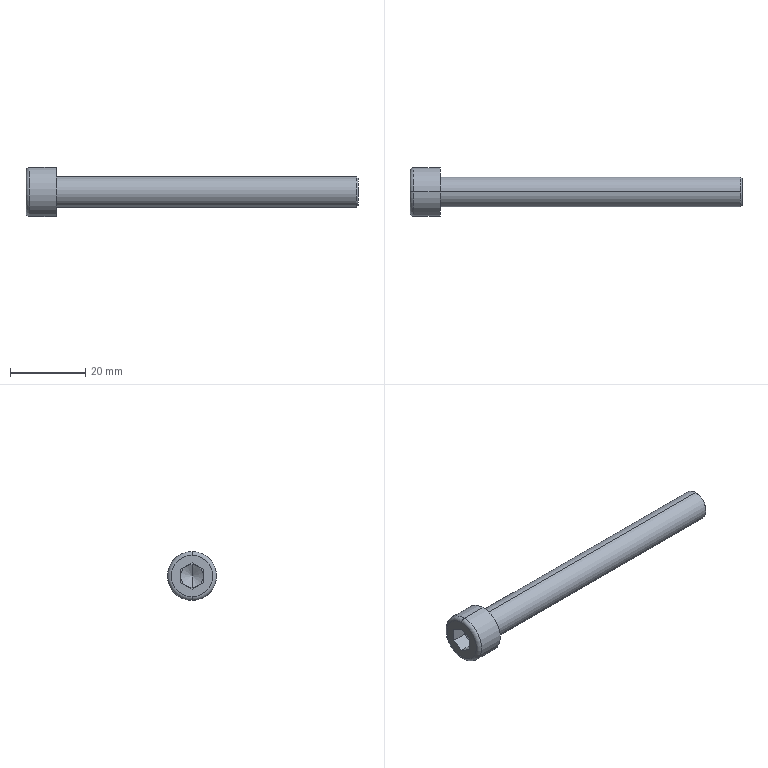Component | SolidWorks | M8X80-2 | 1 solid | 25 faces | box 88 x 13 x 13 mm | volume 4932 mm3 | plane 15 | cone 4 | cylinder 4 | torus 2 | commonest cylinder face diameters 8 x2 13 x2
build123d program:
from build123d import *

# Parameters (mm, degrees)
SKETCH1_R           = 6.5
BASEHEAD_DEPTH      = 8
SKETCH2_R           = 4
BASEBODY_DEPTH      = 80
HEXAGONSOCKET_DEPTH = 4
TOPFILLET_R         = 1
CHAMFER1_SIZE       = 0.4


with BuildPart() as part:
    # Sketch1 → BaseHead (new body)
    with BuildSketch(Plane(origin=(0, 0, 0), x_dir=(0, 0, -1), z_dir=(1, 0, 0))):
        Circle(SKETCH1_R)
    extrude(amount=BASEHEAD_DEPTH)

    # Sketch2 → BaseBody (add)
    with BuildSketch(Plane(origin=(8, 0, 0), x_dir=(0, 0, -1), z_dir=(1, 0, 0))):
        Circle(SKETCH2_R)
    extrude(amount=BASEBODY_DEPTH)

    # Sketch3 → HexagonSocket (cut)
    with BuildSketch(Plane(origin=(0, 0, 0), x_dir=(0, 0, -1), z_dir=(1, 0, 0))):
        Polygon((3.464, 0), (1.732, 3), (-1.732, 3), (-3.464, 0), (-1.732, -3), (1.732, -3), align=None)
    extrude(amount=HEXAGONSOCKET_DEPTH, mode=Mode.SUBTRACT)

    # Sketch4 → Cut-Revolve1 (revolve, cut)
    with BuildSketch(Plane(origin=(-4.196, 0.75, 0), x_dir=(-1, 0, 0), z_dir=(0, 0, 1)), mode=Mode.PRIVATE) as cut_revolve1_sk:
        Polygon((-8.196, 3.75), (-9.928, 0.75), (-8.196, 0.75), align=None)
    revolve(cut_revolve1_sk.sketch.rotate(Axis((0.839, 0, 0), (-1, 0, 0)), 90), axis=Axis((0.839, 0, 0), (-1, 0, 0)), mode=Mode.SUBTRACT)

    # TopFillet
    topfillet_edges = [part.edges().sort_by_distance(p)[0] for p in [
        (0, 0, 6.5),
    ]]
    fillet(topfillet_edges, radius=TOPFILLET_R)

    # Chamfer1
    chamfer1_edges = [part.edges().sort_by_distance(p)[0] for p in [
        (88, 0, 4),
    ]]
    chamfer(chamfer1_edges, length=CHAMFER1_SIZE)


solid = part.part

# Placed as in the assembly
solid = solid.moved(Location((-198, 1239.5, 160), (0, 0, 0)))
STEP:
#1=COLOUR_RGB('',0.7922,0.8196,0.9333);
#2=FILL_AREA_STYLE_COLOUR('',#1);
#3=FILL_AREA_STYLE('',(#2));
#4=SURFACE_STYLE_FILL_AREA(#3);
#5=SURFACE_SIDE_STYLE('',(#4));
#6=SURFACE_STYLE_USAGE(.BOTH.,#5);
#7=PRESENTATION_STYLE_ASSIGNMENT((#6));
#8=CARTESIAN_POINT('',(-4.331,48.799,6.157));
#9=VERTEX_POINT('',#8);
#10=CARTESIAN_POINT('',(-4.331,48.799,6.441));
#11=VERTEX_POINT('',#10);
#12=CARTESIAN_POINT('',(-4.331,48.799,6.299));
#13=DIRECTION('',(1.,0.,0.));
#14=DIRECTION('',(0.,0.,-1.));
#15=AXIS2_PLACEMENT_3D('',#12,#13,#14);
#16=CIRCLE('',#15,0.1417);
#17=EDGE_CURVE('',#9,#11,#16,.T.);
#18=ORIENTED_EDGE('',*,*,#17,.F.);
#19=CARTESIAN_POINT('',(-4.346,48.799,6.142));
#20=VERTEX_POINT('',#19);
#21=CARTESIAN_POINT('',(-4.331,48.799,6.157));
#22=DIRECTION('',(-0.7071,0.,-0.7071));
#23=VECTOR('',#22,39.37);
#24=LINE('',#21,#23);
#25=EDGE_CURVE('',#9,#20,#24,.T.);
#26=ORIENTED_EDGE('',*,*,#25,.T.);
#27=CARTESIAN_POINT('',(-4.346,48.799,6.457));
#28=VERTEX_POINT('',#27);
#29=CARTESIAN_POINT('',(-4.346,48.799,6.299));
#30=DIRECTION('',(-1.,0.,0.));
#31=DIRECTION('',(0.,0.,-1.));
#32=AXIS2_PLACEMENT_3D('',#29,#30,#31);
#33=CIRCLE('',#32,0.1575);
#34=EDGE_CURVE('',#28,#20,#33,.T.);
#35=ORIENTED_EDGE('',*,*,#34,.F.);
#36=CARTESIAN_POINT('',(-4.331,48.799,6.441));
#37=DIRECTION('',(-0.7071,0.,0.7071));
#38=VECTOR('',#37,39.37);
#39=LINE('',#36,#38);
#40=EDGE_CURVE('',#11,#28,#39,.T.);
#41=ORIENTED_EDGE('',*,*,#40,.F.);
#42=EDGE_LOOP('',(#18,#26,#35,#41));
#43=FACE_OUTER_BOUND('',#42,.T.);
#44=CARTESIAN_POINT('',(-4.331,48.799,6.299));
#45=DIRECTION('',(-1.,0.,0.));
#46=DIRECTION('',(0.,0.,1.));
#47=AXIS2_PLACEMENT_3D('',#44,#45,#46);
#48=CONICAL_SURFACE('',#47,0.1417,0.7854);
#49=ADVANCED_FACE('',(#43),#48,.T.);
#50=CARTESIAN_POINT('',(-7.795,48.799,6.516));
#51=VERTEX_POINT('',#50);
#52=CARTESIAN_POINT('',(-7.795,48.799,6.083));
#53=VERTEX_POINT('',#52);
#54=CARTESIAN_POINT('',(-7.795,48.799,6.299));
#55=DIRECTION('',(-1.,0.,0.));
#56=DIRECTION('',(0.,0.,-1.));
#57=AXIS2_PLACEMENT_3D('',#54,#55,#56);
#58=CIRCLE('',#57,0.2165);
#59=EDGE_CURVE('',#51,#53,#58,.T.);
#60=ORIENTED_EDGE('',*,*,#59,.F.);
#61=CARTESIAN_POINT('',(-7.756,48.799,6.555));
#62=VERTEX_POINT('',#61);
#63=CARTESIAN_POINT('',(-7.756,48.799,6.516));
#64=DIRECTION('',(0.,1.,-0.));
#65=DIRECTION('',(0.,0.,1.));
#66=AXIS2_PLACEMENT_3D('',#63,#64,#65);
#67=CIRCLE('',#66,0.03937);
#68=EDGE_CURVE('',#51,#62,#67,.T.);
#69=ORIENTED_EDGE('',*,*,#68,.T.);
#70=CARTESIAN_POINT('',(-7.756,48.799,6.043));
#71=VERTEX_POINT('',#70);
#72=CARTESIAN_POINT('',(-7.756,48.799,6.299));
#73=DIRECTION('',(1.,0.,0.));
#74=DIRECTION('',(0.,0.,-1.));
#75=AXIS2_PLACEMENT_3D('',#72,#73,#74);
#76=CIRCLE('',#75,0.2559);
#77=EDGE_CURVE('',#71,#62,#76,.T.);
#78=ORIENTED_EDGE('',*,*,#77,.F.);
#79=CARTESIAN_POINT('',(-7.756,48.799,6.083));
#80=DIRECTION('',(0.,-1.,0.));
#81=DIRECTION('',(0.,0.,-1.));
#82=AXIS2_PLACEMENT_3D('',#79,#80,#81);
#83=CIRCLE('',#82,0.03937);
#84=EDGE_CURVE('',#53,#71,#83,.T.);
#85=ORIENTED_EDGE('',*,*,#84,.F.);
#86=EDGE_LOOP('',(#60,#69,#78,#85));
#87=FACE_OUTER_BOUND('',#86,.T.);
#88=CARTESIAN_POINT('',(-7.756,48.799,6.299));
#89=DIRECTION('',(1.,0.,0.));
#90=DIRECTION('',(0.,0.,-1.));
#91=AXIS2_PLACEMENT_3D('',#88,#89,#90);
#92=TOROIDAL_SURFACE('',#91,0.2165,0.03937);
#93=ADVANCED_FACE('',(#87),#92,.T.);
#94=CARTESIAN_POINT('',(-7.57,48.799,6.299));
#95=VERTEX_POINT('',#94);
#96=CARTESIAN_POINT('',(-7.638,48.799,6.417));
#97=VERTEX_POINT('',#96);
#98=CARTESIAN_POINT('',(-7.638,48.799,6.417));
#99=DIRECTION('',(-0.5,0.,0.866));
#100=VECTOR('',#99,39.37);
#101=LINE('',#98,#100);
#102=EDGE_CURVE('',#95,#97,#101,.T.);
#103=ORIENTED_EDGE('',*,*,#102,.F.);
#104=CARTESIAN_POINT('',(-7.638,48.799,6.181));
#105=VERTEX_POINT('',#104);
#106=CARTESIAN_POINT('',(-7.638,48.799,6.181));
#107=DIRECTION('',(-0.5,0.,-0.866));
#108=VECTOR('',#107,39.37);
#109=LINE('',#106,#108);
#110=EDGE_CURVE('',#95,#105,#109,.T.);
#111=ORIENTED_EDGE('',*,*,#110,.T.);
#112=CARTESIAN_POINT('',(-7.638,48.74,6.197));
#113=VERTEX_POINT('',#112);
#114=CARTESIAN_POINT('',(-7.638,48.799,6.299));
#115=DIRECTION('',(-1.,0.,0.));
#116=DIRECTION('',(0.,0.,-1.));
#117=AXIS2_PLACEMENT_3D('',#114,#115,#116);
#118=CIRCLE('',#117,0.1181);
#119=EDGE_CURVE('',#105,#113,#118,.T.);
#120=ORIENTED_EDGE('',*,*,#119,.T.);
#121=CARTESIAN_POINT('',(-7.638,48.681,6.299));
#122=VERTEX_POINT('',#121);
#123=CARTESIAN_POINT('',(-7.638,48.799,6.299));
#124=DIRECTION('',(-1.,0.,0.));
#125=DIRECTION('',(0.,0.,-1.));
#126=AXIS2_PLACEMENT_3D('',#123,#124,#125);
#127=CIRCLE('',#126,0.1181);
#128=EDGE_CURVE('',#113,#122,#127,.T.);
#129=ORIENTED_EDGE('',*,*,#128,.T.);
#130=CARTESIAN_POINT('',(-7.638,48.74,6.401));
#131=VERTEX_POINT('',#130);
#132=CARTESIAN_POINT('',(-7.638,48.799,6.299));
#133=DIRECTION('',(-1.,0.,0.));
#134=DIRECTION('',(0.,0.,-1.));
#135=AXIS2_PLACEMENT_3D('',#132,#133,#134);
#136=CIRCLE('',#135,0.1181);
#137=EDGE_CURVE('',#122,#131,#136,.T.);
#138=ORIENTED_EDGE('',*,*,#137,.T.);
#139=CARTESIAN_POINT('',(-7.638,48.799,6.299));
#140=DIRECTION('',(-1.,0.,0.));
#141=DIRECTION('',(0.,0.,-1.));
#142=AXIS2_PLACEMENT_3D('',#139,#140,#141);
#143=CIRCLE('',#142,0.1181);
#144=EDGE_CURVE('',#131,#97,#143,.T.);
#145=ORIENTED_EDGE('',*,*,#144,.T.);
#146=EDGE_LOOP('',(#103,#111,#120,#129,#138,#145));
#147=FACE_OUTER_BOUND('',#146,.T.);
#148=CARTESIAN_POINT('',(-7.638,48.799,6.299));
#149=DIRECTION('',(-1.,0.,0.));
#150=DIRECTION('',(0.,0.,1.));
#151=AXIS2_PLACEMENT_3D('',#148,#149,#150);
#152=CONICAL_SURFACE('',#151,0.1181,1.047);
#153=ADVANCED_FACE('',(#147),#152,.F.);
#154=ORIENTED_EDGE('',*,*,#34,.T.);
#155=CARTESIAN_POINT('',(-7.48,48.799,6.142));
#156=VERTEX_POINT('',#155);
#157=CARTESIAN_POINT('',(-4.331,48.799,6.142));
#158=DIRECTION('',(-1.,0.,0.));
#159=VECTOR('',#158,39.37);
#160=LINE('',#157,#159);
#161=EDGE_CURVE('',#20,#156,#160,.T.);
#162=ORIENTED_EDGE('',*,*,#161,.T.);
#163=CARTESIAN_POINT('',(-7.48,48.799,6.457));
#164=VERTEX_POINT('',#163);
#165=CARTESIAN_POINT('',(-7.48,48.799,6.299));
#166=DIRECTION('',(1.,0.,0.));
#167=DIRECTION('',(0.,0.,-1.));
#168=AXIS2_PLACEMENT_3D('',#165,#166,#167);
#169=CIRCLE('',#168,0.1575);
#170=EDGE_CURVE('',#156,#164,#169,.T.);
#171=ORIENTED_EDGE('',*,*,#170,.T.);
#172=CARTESIAN_POINT('',(-4.331,48.799,6.457));
#173=DIRECTION('',(-1.,0.,0.));
#174=VECTOR('',#173,39.37);
#175=LINE('',#172,#174);
#176=EDGE_CURVE('',#28,#164,#175,.T.);
#177=ORIENTED_EDGE('',*,*,#176,.F.);
#178=EDGE_LOOP('',(#154,#162,#171,#177));
#179=FACE_OUTER_BOUND('',#178,.T.);
#180=CARTESIAN_POINT('',(-4.331,48.799,6.299));
#181=DIRECTION('',(-1.,0.,0.));
#182=DIRECTION('',(0.,0.,1.));
#183=AXIS2_PLACEMENT_3D('',#180,#181,#182);
#184=CYLINDRICAL_SURFACE('',#183,0.1575);
#185=ADVANCED_FACE('',(#179),#184,.T.);
#186=CARTESIAN_POINT('',(-7.48,48.799,6.043));
#187=VERTEX_POINT('',#186);
#188=CARTESIAN_POINT('',(-7.48,48.799,6.555));
#189=VERTEX_POINT('',#188);
#190=CARTESIAN_POINT('',(-7.48,48.799,6.299));
#191=DIRECTION('',(1.,0.,0.));
#192=DIRECTION('',(0.,0.,-1.));
#193=AXIS2_PLACEMENT_3D('',#190,#191,#192);
#194=CIRCLE('',#193,0.2559);
#195=EDGE_CURVE('',#187,#189,#194,.T.);
#196=ORIENTED_EDGE('',*,*,#195,.F.);
#197=CARTESIAN_POINT('',(-7.48,48.799,6.043));
#198=DIRECTION('',(-1.,0.,0.));
#199=VECTOR('',#198,39.37);
#200=LINE('',#197,#199);
#201=EDGE_CURVE('',#187,#71,#200,.T.);
#202=ORIENTED_EDGE('',*,*,#201,.T.);
#203=ORIENTED_EDGE('',*,*,#77,.T.);
#204=CARTESIAN_POINT('',(-7.48,48.799,6.555));
#205=DIRECTION('',(-1.,0.,0.));
#206=VECTOR('',#205,39.37);
#207=LINE('',#204,#206);
#208=EDGE_CURVE('',#189,#62,#207,.T.);
#209=ORIENTED_EDGE('',*,*,#208,.F.);
#210=EDGE_LOOP('',(#196,#202,#203,#209));
#211=FACE_OUTER_BOUND('',#210,.T.);
#212=CARTESIAN_POINT('',(-7.48,48.799,6.299));
#213=DIRECTION('',(-1.,0.,0.));
#214=DIRECTION('',(0.,0.,1.));
#215=AXIS2_PLACEMENT_3D('',#212,#213,#214);
#216=CYLINDRICAL_SURFACE('',#215,0.2559);
#217=ADVANCED_FACE('',(#211),#216,.T.);
#218=ORIENTED_EDGE('',*,*,#128,.F.);
#219=CARTESIAN_POINT('',(-7.638,48.681,6.231));
#220=VERTEX_POINT('',#219);
#221=CARTESIAN_POINT('',(-7.638,48.681,6.231));
#222=DIRECTION('',(0.,0.866,-0.5));
#223=VECTOR('',#222,39.37);
#224=LINE('',#221,#223);
#225=EDGE_CURVE('',#220,#113,#224,.T.);
#226=ORIENTED_EDGE('',*,*,#225,.F.);
#227=CARTESIAN_POINT('',(-7.638,48.681,6.367));
#228=DIRECTION('',(0.,-0.,-1.));
#229=VECTOR('',#228,39.37);
#230=LINE('',#227,#229);
#231=EDGE_CURVE('',#122,#220,#230,.T.);
#232=ORIENTED_EDGE('',*,*,#231,.F.);
#233=EDGE_LOOP('',(#218,#226,#232));
#234=FACE_OUTER_BOUND('',#233,.T.);
#235=CARTESIAN_POINT('',(-7.638,48.799,6.163));
#236=DIRECTION('',(1.,0.,0.));
#237=DIRECTION('',(0.,0.,-1.));
#238=AXIS2_PLACEMENT_3D('',#235,#236,#237);
#239=PLANE('',#238);
#240=ADVANCED_FACE('',(#234),#239,.F.);
#241=ORIENTED_EDGE('',*,*,#137,.F.);
#242=CARTESIAN_POINT('',(-7.638,48.681,6.367));
#243=VERTEX_POINT('',#242);
#244=CARTESIAN_POINT('',(-7.638,48.681,6.367));
#245=DIRECTION('',(0.,-0.,-1.));
#246=VECTOR('',#245,39.37);
#247=LINE('',#244,#246);
#248=EDGE_CURVE('',#243,#122,#247,.T.);
#249=ORIENTED_EDGE('',*,*,#248,.F.);
#250=CARTESIAN_POINT('',(-7.638,48.799,6.436));
#251=DIRECTION('',(0.,-0.866,-0.5));
#252=VECTOR('',#251,39.37);
#253=LINE('',#250,#252);
#254=EDGE_CURVE('',#131,#243,#253,.T.);
#255=ORIENTED_EDGE('',*,*,#254,.F.);
#256=EDGE_LOOP('',(#241,#249,#255));
#257=FACE_OUTER_BOUND('',#256,.T.);
#258=CARTESIAN_POINT('',(-7.638,48.799,6.163));
#259=DIRECTION('',(1.,0.,0.));
#260=DIRECTION('',(0.,0.,-1.));
#261=AXIS2_PLACEMENT_3D('',#258,#259,#260);
#262=PLANE('',#261);
#263=ADVANCED_FACE('',(#257),#262,.F.);
#264=ORIENTED_EDGE('',*,*,#144,.F.);
#265=CARTESIAN_POINT('',(-7.638,48.799,6.436));
#266=VERTEX_POINT('',#265);
#267=CARTESIAN_POINT('',(-7.638,48.799,6.436));
#268=DIRECTION('',(0.,-0.866,-0.5));
#269=VECTOR('',#268,39.37);
#270=LINE('',#267,#269);
#271=EDGE_CURVE('',#266,#131,#270,.T.);
#272=ORIENTED_EDGE('',*,*,#271,.F.);
#273=CARTESIAN_POINT('',(-7.638,48.858,6.401));
#274=VERTEX_POINT('',#273);
#275=CARTESIAN_POINT('',(-7.638,48.917,6.367));
#276=DIRECTION('',(0.,-0.866,0.5));
#277=VECTOR('',#276,39.37);
#278=LINE('',#275,#277);
#279=EDGE_CURVE('',#274,#266,#278,.T.);
#280=ORIENTED_EDGE('',*,*,#279,.F.);
#281=CARTESIAN_POINT('',(-7.638,48.799,6.299));
#282=DIRECTION('',(-1.,0.,0.));
#283=DIRECTION('',(0.,0.,-1.));
#284=AXIS2_PLACEMENT_3D('',#281,#282,#283);
#285=CIRCLE('',#284,0.1181);
#286=EDGE_CURVE('',#97,#274,#285,.T.);
#287=ORIENTED_EDGE('',*,*,#286,.F.);
#288=EDGE_LOOP('',(#264,#272,#280,#287));
#289=FACE_OUTER_BOUND('',#288,.T.);
#290=CARTESIAN_POINT('',(-7.638,48.799,6.163));
#291=DIRECTION('',(1.,0.,0.));
#292=DIRECTION('',(0.,0.,-1.));
#293=AXIS2_PLACEMENT_3D('',#290,#291,#292);
#294=PLANE('',#293);
#295=ADVANCED_FACE('',(#289),#294,.F.);
#296=CARTESIAN_POINT('',(-7.638,48.917,6.299));
#297=VERTEX_POINT('',#296);
#298=CARTESIAN_POINT('',(-7.638,48.799,6.299));
#299=DIRECTION('',(-1.,0.,0.));
#300=DIRECTION('',(0.,0.,-1.));
#301=AXIS2_PLACEMENT_3D('',#298,#299,#300);
#302=CIRCLE('',#301,0.1181);
#303=EDGE_CURVE('',#274,#297,#302,.T.);
#304=ORIENTED_EDGE('',*,*,#303,.F.);
#305=CARTESIAN_POINT('',(-7.638,48.917,6.367));
#306=VERTEX_POINT('',#305);
#307=CARTESIAN_POINT('',(-7.638,48.917,6.367));
#308=DIRECTION('',(0.,-0.866,0.5));
#309=VECTOR('',#308,39.37);
#310=LINE('',#307,#309);
#311=EDGE_CURVE('',#306,#274,#310,.T.);
#312=ORIENTED_EDGE('',*,*,#311,.F.);
#313=CARTESIAN_POINT('',(-7.638,48.917,6.231));
#314=DIRECTION('',(0.,0.,1.));
#315=VECTOR('',#314,39.37);
#316=LINE('',#313,#315);
#317=EDGE_CURVE('',#297,#306,#316,.T.);
#318=ORIENTED_EDGE('',*,*,#317,.F.);
#319=EDGE_LOOP('',(#304,#312,#318));
#320=FACE_OUTER_BOUND('',#319,.T.);
#321=CARTESIAN_POINT('',(-7.638,48.799,6.163));
#322=DIRECTION('',(1.,0.,0.));
#323=DIRECTION('',(0.,0.,-1.));
#324=AXIS2_PLACEMENT_3D('',#321,#322,#323);
#325=PLANE('',#324);
#326=ADVANCED_FACE('',(#320),#325,.F.);
#327=CARTESIAN_POINT('',(-7.638,48.858,6.197));
#328=VERTEX_POINT('',#327);
#329=CARTESIAN_POINT('',(-7.638,48.799,6.299));
#330=DIRECTION('',(1.,0.,0.));
#331=DIRECTION('',(0.,0.,-1.));
#332=AXIS2_PLACEMENT_3D('',#329,#330,#331);
#333=CIRCLE('',#332,0.1181);
#334=EDGE_CURVE('',#328,#297,#333,.T.);
#335=ORIENTED_EDGE('',*,*,#334,.T.);
#336=CARTESIAN_POINT('',(-7.638,48.917,6.231));
#337=VERTEX_POINT('',#336);
#338=CARTESIAN_POINT('',(-7.638,48.917,6.231));
#339=DIRECTION('',(0.,0.,1.));
#340=VECTOR('',#339,39.37);
#341=LINE('',#338,#340);
#342=EDGE_CURVE('',#337,#297,#341,.T.);
#343=ORIENTED_EDGE('',*,*,#342,.F.);
#344=CARTESIAN_POINT('',(-7.638,48.799,6.163));
#345=DIRECTION('',(0.,0.866,0.5));
#346=VECTOR('',#345,39.37);
#347=LINE('',#344,#346);
#348=EDGE_CURVE('',#328,#337,#347,.T.);
#349=ORIENTED_EDGE('',*,*,#348,.F.);
#350=EDGE_LOOP('',(#335,#343,#349));
#351=FACE_OUTER_BOUND('',#350,.T.);
#352=CARTESIAN_POINT('',(-7.638,48.799,6.163));
#353=DIRECTION('',(1.,0.,0.));
#354=DIRECTION('',(0.,0.,-1.));
#355=AXIS2_PLACEMENT_3D('',#352,#353,#354);
#356=PLANE('',#355);
#357=ADVANCED_FACE('',(#351),#356,.F.);
#358=CARTESIAN_POINT('',(-7.638,48.799,6.299));
#359=DIRECTION('',(-1.,0.,0.));
#360=DIRECTION('',(0.,0.,-1.));
#361=AXIS2_PLACEMENT_3D('',#358,#359,#360);
#362=CIRCLE('',#361,0.1181);
#363=EDGE_CURVE('',#328,#105,#362,.T.);
#364=ORIENTED_EDGE('',*,*,#363,.F.);
#365=CARTESIAN_POINT('',(-7.638,48.799,6.163));
#366=VERTEX_POINT('',#365);
#367=CARTESIAN_POINT('',(-7.638,48.799,6.163));
#368=DIRECTION('',(0.,0.866,0.5));
#369=VECTOR('',#368,39.37);
#370=LINE('',#367,#369);
#371=EDGE_CURVE('',#366,#328,#370,.T.);
#372=ORIENTED_EDGE('',*,*,#371,.F.);
#373=CARTESIAN_POINT('',(-7.638,48.681,6.231));
#374=DIRECTION('',(0.,0.866,-0.5));
#375=VECTOR('',#374,39.37);
#376=LINE('',#373,#375);
#377=EDGE_CURVE('',#113,#366,#376,.T.);
#378=ORIENTED_EDGE('',*,*,#377,.F.);
#379=ORIENTED_EDGE('',*,*,#119,.F.);
#380=EDGE_LOOP('',(#364,#372,#378,#379));
#381=FACE_OUTER_BOUND('',#380,.T.);
#382=CARTESIAN_POINT('',(-7.638,48.799,6.163));
#383=DIRECTION('',(1.,0.,0.));
#384=DIRECTION('',(0.,0.,-1.));
#385=AXIS2_PLACEMENT_3D('',#382,#383,#384);
#386=PLANE('',#385);
#387=ADVANCED_FACE('',(#381),#386,.F.);
#388=CARTESIAN_POINT('',(-7.795,48.799,6.299));
#389=DIRECTION('',(-1.,0.,0.));
#390=DIRECTION('',(0.,0.,-1.));
#391=AXIS2_PLACEMENT_3D('',#388,#389,#390);
#392=CIRCLE('',#391,0.2165);
#393=EDGE_CURVE('',#53,#51,#392,.T.);
#394=ORIENTED_EDGE('',*,*,#393,.T.);
#395=ORIENTED_EDGE('',*,*,#59,.T.);
#396=EDGE_LOOP('',(#394,#395));
#397=FACE_OUTER_BOUND('',#396,.T.);
#398=CARTESIAN_POINT('',(-7.795,48.681,6.231));
#399=VERTEX_POINT('',#398);
#400=CARTESIAN_POINT('',(-7.795,48.799,6.163));
#401=VERTEX_POINT('',#400);
#402=CARTESIAN_POINT('',(-7.795,48.681,6.231));
#403=DIRECTION('',(0.,0.866,-0.5));
#404=VECTOR('',#403,39.37);
#405=LINE('',#402,#404);
#406=EDGE_CURVE('',#399,#401,#405,.T.);
#407=ORIENTED_EDGE('',*,*,#406,.T.);
#408=CARTESIAN_POINT('',(-7.795,48.917,6.231));
#409=VERTEX_POINT('',#408);
#410=CARTESIAN_POINT('',(-7.795,48.799,6.163));
#411=DIRECTION('',(0.,0.866,0.5));
#412=VECTOR('',#411,39.37);
#413=LINE('',#410,#412);
#414=EDGE_CURVE('',#401,#409,#413,.T.);
#415=ORIENTED_EDGE('',*,*,#414,.T.);
#416=CARTESIAN_POINT('',(-7.795,48.917,6.367));
#417=VERTEX_POINT('',#416);
#418=CARTESIAN_POINT('',(-7.795,48.917,6.231));
#419=DIRECTION('',(0.,0.,1.));
#420=VECTOR('',#419,39.37);
#421=LINE('',#418,#420);
#422=EDGE_CURVE('',#409,#417,#421,.T.);
#423=ORIENTED_EDGE('',*,*,#422,.T.);
#424=CARTESIAN_POINT('',(-7.795,48.799,6.436));
#425=VERTEX_POINT('',#424);
#426=CARTESIAN_POINT('',(-7.795,48.917,6.367));
#427=DIRECTION('',(0.,-0.866,0.5));
#428=VECTOR('',#427,39.37);
#429=LINE('',#426,#428);
#430=EDGE_CURVE('',#417,#425,#429,.T.);
#431=ORIENTED_EDGE('',*,*,#430,.T.);
#432=CARTESIAN_POINT('',(-7.795,48.681,6.367));
#433=VERTEX_POINT('',#432);
#434=CARTESIAN_POINT('',(-7.795,48.799,6.436));
#435=DIRECTION('',(0.,-0.866,-0.5));
#436=VECTOR('',#435,39.37);
#437=LINE('',#434,#436);
#438=EDGE_CURVE('',#425,#433,#437,.T.);
#439=ORIENTED_EDGE('',*,*,#438,.T.);
#440=CARTESIAN_POINT('',(-7.795,48.681,6.367));
#441=DIRECTION('',(0.,-0.,-1.));
#442=VECTOR('',#441,39.37);
#443=LINE('',#440,#442);
#444=EDGE_CURVE('',#433,#399,#443,.T.);
#445=ORIENTED_EDGE('',*,*,#444,.T.);
#446=EDGE_LOOP('',(#407,#415,#423,#431,#439,#445));
#447=FACE_BOUND('',#446,.T.);
#448=CARTESIAN_POINT('',(-7.795,48.799,6.299));
#449=DIRECTION('',(1.,0.,0.));
#450=DIRECTION('',(0.,0.,-1.));
#451=AXIS2_PLACEMENT_3D('',#448,#449,#450);
#452=PLANE('',#451);
#453=ADVANCED_FACE('',(#397,#447),#452,.F.);
#454=CARTESIAN_POINT('',(-7.48,48.799,6.299));
#455=DIRECTION('',(1.,0.,0.));
#456=DIRECTION('',(0.,0.,-1.));
#457=AXIS2_PLACEMENT_3D('',#454,#455,#456);
#458=CIRCLE('',#457,0.2559);
#459=EDGE_CURVE('',#189,#187,#458,.T.);
#460=ORIENTED_EDGE('',*,*,#459,.T.);
#461=ORIENTED_EDGE('',*,*,#195,.T.);
#462=EDGE_LOOP('',(#460,#461));
#463=FACE_OUTER_BOUND('',#462,.T.);
#464=CARTESIAN_POINT('',(-7.48,48.799,6.299));
#465=DIRECTION('',(1.,0.,0.));
#466=DIRECTION('',(0.,0.,-1.));
#467=AXIS2_PLACEMENT_3D('',#464,#465,#466);
#468=CIRCLE('',#467,0.1575);
#469=EDGE_CURVE('',#164,#156,#468,.T.);
#470=ORIENTED_EDGE('',*,*,#469,.F.);
#471=ORIENTED_EDGE('',*,*,#170,.F.);
#472=EDGE_LOOP('',(#470,#471));
#473=FACE_BOUND('',#472,.T.);
#474=CARTESIAN_POINT('',(-7.48,48.799,6.299));
#475=DIRECTION('',(1.,0.,0.));
#476=DIRECTION('',(0.,0.,-1.));
#477=AXIS2_PLACEMENT_3D('',#474,#475,#476);
#478=PLANE('',#477);
#479=ADVANCED_FACE('',(#463,#473),#478,.T.);
#480=ORIENTED_EDGE('',*,*,#201,.F.);
#481=ORIENTED_EDGE('',*,*,#459,.F.);
#482=ORIENTED_EDGE('',*,*,#208,.T.);
#483=CARTESIAN_POINT('',(-7.756,48.799,6.299));
#484=DIRECTION('',(1.,0.,0.));
#485=DIRECTION('',(0.,0.,-1.));
#486=AXIS2_PLACEMENT_3D('',#483,#484,#485);
#487=CIRCLE('',#486,0.2559);
#488=EDGE_CURVE('',#62,#71,#487,.T.);
#489=ORIENTED_EDGE('',*,*,#488,.T.);
#490=EDGE_LOOP('',(#480,#481,#482,#489));
#491=FACE_OUTER_BOUND('',#490,.T.);
#492=CARTESIAN_POINT('',(-7.48,48.799,6.299));
#493=DIRECTION('',(-1.,0.,0.));
#494=DIRECTION('',(0.,0.,1.));
#495=AXIS2_PLACEMENT_3D('',#492,#493,#494);
#496=CYLINDRICAL_SURFACE('',#495,0.2559);
#497=ADVANCED_FACE('',(#491),#496,.T.);
#498=ORIENTED_EDGE('',*,*,#161,.F.);
#499=CARTESIAN_POINT('',(-4.346,48.799,6.299));
#500=DIRECTION('',(-1.,0.,0.));
#501=DIRECTION('',(0.,0.,-1.));
#502=AXIS2_PLACEMENT_3D('',#499,#500,#501);
#503=CIRCLE('',#502,0.1575);
#504=EDGE_CURVE('',#20,#28,#503,.T.);
#505=ORIENTED_EDGE('',*,*,#504,.T.);
#506=ORIENTED_EDGE('',*,*,#176,.T.);
#507=ORIENTED_EDGE('',*,*,#469,.T.);
#508=EDGE_LOOP('',(#498,#505,#506,#507));
#509=FACE_OUTER_BOUND('',#508,.T.);
#510=CARTESIAN_POINT('',(-4.331,48.799,6.299));
#511=DIRECTION('',(-1.,0.,0.));
#512=DIRECTION('',(0.,0.,1.));
#513=AXIS2_PLACEMENT_3D('',#510,#511,#512);
#514=CYLINDRICAL_SURFACE('',#513,0.1575);
#515=ADVANCED_FACE('',(#509),#514,.T.);
#516=CARTESIAN_POINT('',(-4.331,48.799,6.299));
#517=DIRECTION('',(1.,0.,0.));
#518=DIRECTION('',(0.,0.,-1.));
#519=AXIS2_PLACEMENT_3D('',#516,#517,#518);
#520=CIRCLE('',#519,0.1417);
#521=EDGE_CURVE('',#11,#9,#520,.T.);
#522=ORIENTED_EDGE('',*,*,#521,.T.);
#523=ORIENTED_EDGE('',*,*,#17,.T.);
#524=EDGE_LOOP('',(#522,#523));
#525=FACE_OUTER_BOUND('',#524,.T.);
#526=CARTESIAN_POINT('',(-4.331,48.799,6.299));
#527=DIRECTION('',(1.,0.,0.));
#528=DIRECTION('',(0.,0.,-1.));
#529=AXIS2_PLACEMENT_3D('',#526,#527,#528);
#530=PLANE('',#529);
#531=ADVANCED_FACE('',(#525),#530,.T.);
#532=ORIENTED_EDGE('',*,*,#406,.F.);
#533=CARTESIAN_POINT('',(-7.638,48.681,6.231));
#534=DIRECTION('',(-1.,0.,0.));
#535=VECTOR('',#534,39.37);
#536=LINE('',#533,#535);
#537=EDGE_CURVE('',#220,#399,#536,.T.);
#538=ORIENTED_EDGE('',*,*,#537,.F.);
#539=ORIENTED_EDGE('',*,*,#225,.T.);
#540=ORIENTED_EDGE('',*,*,#377,.T.);
#541=CARTESIAN_POINT('',(-7.638,48.799,6.163));
#542=DIRECTION('',(-1.,0.,0.));
#543=VECTOR('',#542,39.37);
#544=LINE('',#541,#543);
#545=EDGE_CURVE('',#366,#401,#544,.T.);
#546=ORIENTED_EDGE('',*,*,#545,.T.);
#547=EDGE_LOOP('',(#532,#538,#539,#540,#546));
#548=FACE_OUTER_BOUND('',#547,.T.);
#549=CARTESIAN_POINT('',(-7.638,48.681,6.231));
#550=DIRECTION('',(0.,0.5,0.866));
#551=DIRECTION('',(0.,-0.866,0.5));
#552=AXIS2_PLACEMENT_3D('',#549,#550,#551);
#553=PLANE('',#552);
#554=ADVANCED_FACE('',(#548),#553,.T.);
#555=ORIENTED_EDGE('',*,*,#414,.F.);
#556=ORIENTED_EDGE('',*,*,#545,.F.);
#557=ORIENTED_EDGE('',*,*,#371,.T.);
#558=ORIENTED_EDGE('',*,*,#348,.T.);
#559=CARTESIAN_POINT('',(-7.638,48.917,6.231));
#560=DIRECTION('',(-1.,0.,0.));
#561=VECTOR('',#560,39.37);
#562=LINE('',#559,#561);
#563=EDGE_CURVE('',#337,#409,#562,.T.);
#564=ORIENTED_EDGE('',*,*,#563,.T.);
#565=EDGE_LOOP('',(#555,#556,#557,#558,#564));
#566=FACE_OUTER_BOUND('',#565,.T.);
#567=CARTESIAN_POINT('',(-7.638,48.799,6.163));
#568=DIRECTION('',(0.,-0.5,0.866));
#569=DIRECTION('',(0.,-0.866,-0.5));
#570=AXIS2_PLACEMENT_3D('',#567,#568,#569);
#571=PLANE('',#570);
#572=ADVANCED_FACE('',(#566),#571,.T.);
#573=ORIENTED_EDGE('',*,*,#422,.F.);
#574=ORIENTED_EDGE('',*,*,#563,.F.);
#575=ORIENTED_EDGE('',*,*,#342,.T.);
#576=ORIENTED_EDGE('',*,*,#317,.T.);
#577=CARTESIAN_POINT('',(-7.638,48.917,6.367));
#578=DIRECTION('',(-1.,0.,0.));
#579=VECTOR('',#578,39.37);
#580=LINE('',#577,#579);
#581=EDGE_CURVE('',#306,#417,#580,.T.);
#582=ORIENTED_EDGE('',*,*,#581,.T.);
#583=EDGE_LOOP('',(#573,#574,#575,#576,#582));
#584=FACE_OUTER_BOUND('',#583,.T.);
#585=CARTESIAN_POINT('',(-7.638,48.917,6.231));
#586=DIRECTION('',(0.,-1.,0.));
#587=DIRECTION('',(0.,0.,-1.));
#588=AXIS2_PLACEMENT_3D('',#585,#586,#587);
#589=PLANE('',#588);
#590=ADVANCED_FACE('',(#584),#589,.T.);
#591=ORIENTED_EDGE('',*,*,#430,.F.);
#592=ORIENTED_EDGE('',*,*,#581,.F.);
#593=ORIENTED_EDGE('',*,*,#311,.T.);
#594=ORIENTED_EDGE('',*,*,#279,.T.);
#595=CARTESIAN_POINT('',(-7.638,48.799,6.436));
#596=DIRECTION('',(-1.,0.,0.));
#597=VECTOR('',#596,39.37);
#598=LINE('',#595,#597);
#599=EDGE_CURVE('',#266,#425,#598,.T.);
#600=ORIENTED_EDGE('',*,*,#599,.T.);
#601=EDGE_LOOP('',(#591,#592,#593,#594,#600));
#602=FACE_OUTER_BOUND('',#601,.T.);
#603=CARTESIAN_POINT('',(-7.638,48.917,6.367));
#604=DIRECTION('',(0.,-0.5,-0.866));
#605=DIRECTION('',(0.,0.866,-0.5));
#606=AXIS2_PLACEMENT_3D('',#603,#604,#605);
#607=PLANE('',#606);
#608=ADVANCED_FACE('',(#602),#607,.T.);
#609=ORIENTED_EDGE('',*,*,#438,.F.);
#610=ORIENTED_EDGE('',*,*,#599,.F.);
#611=ORIENTED_EDGE('',*,*,#271,.T.);
#612=ORIENTED_EDGE('',*,*,#254,.T.);
#613=CARTESIAN_POINT('',(-7.638,48.681,6.367));
#614=DIRECTION('',(-1.,0.,0.));
#615=VECTOR('',#614,39.37);
#616=LINE('',#613,#615);
#617=EDGE_CURVE('',#243,#433,#616,.T.);
#618=ORIENTED_EDGE('',*,*,#617,.T.);
#619=EDGE_LOOP('',(#609,#610,#611,#612,#618));
#620=FACE_OUTER_BOUND('',#619,.T.);
#621=CARTESIAN_POINT('',(-7.638,48.799,6.436));
#622=DIRECTION('',(0.,0.5,-0.866));
#623=DIRECTION('',(0.,0.866,0.5));
#624=AXIS2_PLACEMENT_3D('',#621,#622,#623);
#625=PLANE('',#624);
#626=ADVANCED_FACE('',(#620),#625,.T.);
#627=ORIENTED_EDGE('',*,*,#444,.F.);
#628=ORIENTED_EDGE('',*,*,#617,.F.);
#629=ORIENTED_EDGE('',*,*,#248,.T.);
#630=ORIENTED_EDGE('',*,*,#231,.T.);
#631=ORIENTED_EDGE('',*,*,#537,.T.);
#632=EDGE_LOOP('',(#627,#628,#629,#630,#631));
#633=FACE_OUTER_BOUND('',#632,.T.);
#634=CARTESIAN_POINT('',(-7.638,48.681,6.367));
#635=DIRECTION('',(0.,1.,-0.));
#636=DIRECTION('',(0.,0.,1.));
#637=AXIS2_PLACEMENT_3D('',#634,#635,#636);
#638=PLANE('',#637);
#639=ADVANCED_FACE('',(#633),#638,.T.);
#640=ORIENTED_EDGE('',*,*,#110,.F.);
#641=ORIENTED_EDGE('',*,*,#102,.T.);
#642=ORIENTED_EDGE('',*,*,#286,.T.);
#643=ORIENTED_EDGE('',*,*,#303,.T.);
#644=ORIENTED_EDGE('',*,*,#334,.F.);
#645=ORIENTED_EDGE('',*,*,#363,.T.);
#646=EDGE_LOOP('',(#640,#641,#642,#643,#644,#645));
#647=FACE_OUTER_BOUND('',#646,.T.);
#648=CARTESIAN_POINT('',(-7.638,48.799,6.299));
#649=DIRECTION('',(-1.,0.,0.));
#650=DIRECTION('',(0.,0.,1.));
#651=AXIS2_PLACEMENT_3D('',#648,#649,#650);
#652=CONICAL_SURFACE('',#651,0.1181,1.047);
#653=ADVANCED_FACE('',(#647),#652,.F.);
#654=ORIENTED_EDGE('',*,*,#68,.F.);
#655=ORIENTED_EDGE('',*,*,#393,.F.);
#656=ORIENTED_EDGE('',*,*,#84,.T.);
#657=ORIENTED_EDGE('',*,*,#488,.F.);
#658=EDGE_LOOP('',(#654,#655,#656,#657));
#659=FACE_OUTER_BOUND('',#658,.T.);
#660=CARTESIAN_POINT('',(-7.756,48.799,6.299));
#661=DIRECTION('',(1.,0.,0.));
#662=DIRECTION('',(0.,0.,-1.));
#663=AXIS2_PLACEMENT_3D('',#660,#661,#662);
#664=TOROIDAL_SURFACE('',#663,0.2165,0.03937);
#665=ADVANCED_FACE('',(#659),#664,.T.);
#666=ORIENTED_EDGE('',*,*,#25,.F.);
#667=ORIENTED_EDGE('',*,*,#521,.F.);
#668=ORIENTED_EDGE('',*,*,#40,.T.);
#669=ORIENTED_EDGE('',*,*,#504,.F.);
#670=EDGE_LOOP('',(#666,#667,#668,#669));
#671=FACE_OUTER_BOUND('',#670,.T.);
#672=CARTESIAN_POINT('',(-4.331,48.799,6.299));
#673=DIRECTION('',(-1.,0.,0.));
#674=DIRECTION('',(0.,0.,1.));
#675=AXIS2_PLACEMENT_3D('',#672,#673,#674);
#676=CONICAL_SURFACE('',#675,0.1417,0.7854);
#677=ADVANCED_FACE('',(#671),#676,.T.);
#678=CLOSED_SHELL('',(#49,#93,#153,#185,#217,#240,#263,#295,#326,#357,#387,#453,#479,#497,#515,#531,#554,#572,#590,#608,#626,#639,#653,#665,#677));
#679=MANIFOLD_SOLID_BREP('',#678);
#680=STYLED_ITEM('',(#7),#679);
#681=PRESENTATION_LAYER_ASSIGNMENT('','',(#680));
#682=CARTESIAN_POINT('',(0.,0.,0.));
#683=DIRECTION('',(0.,0.,1.));
#684=DIRECTION('',(1.,0.,0.));
#685=AXIS2_PLACEMENT_3D('',#682,#683,#684);
#686=(LENGTH_UNIT()NAMED_UNIT(*)SI_UNIT($,.METRE.));
#687=LENGTH_MEASURE_WITH_UNIT(LENGTH_MEASURE(0.0254),#686);
#688=DIMENSIONAL_EXPONENTS(1.,0.,0.,0.,0.,0.,0.);
#689=(CONVERSION_BASED_UNIT('',#687)LENGTH_UNIT()NAMED_UNIT(#688));
#690=UNCERTAINTY_MEASURE_WITH_UNIT(LENGTH_MEASURE(0.00001),#689,'','');
#691=(NAMED_UNIT(*)PLANE_ANGLE_UNIT()SI_UNIT($,.RADIAN.));
#692=(NAMED_UNIT(*)SI_UNIT($,.STERADIAN.)SOLID_ANGLE_UNIT());
#693=(GEOMETRIC_REPRESENTATION_CONTEXT(3)GLOBAL_UNCERTAINTY_ASSIGNED_CONTEXT((#690))GLOBAL_UNIT_ASSIGNED_CONTEXT((#689,#691,#692))REPRESENTATION_CONTEXT('',''));
#694=ADVANCED_BREP_SHAPE_REPRESENTATION('',(#679,#685),#693);
#695=(LENGTH_UNIT()NAMED_UNIT(*)SI_UNIT($,.METRE.));
#696=LENGTH_MEASURE_WITH_UNIT(LENGTH_MEASURE(0.0254),#695);
#697=DIMENSIONAL_EXPONENTS(1.,0.,0.,0.,0.,0.,0.);
#698=(CONVERSION_BASED_UNIT('',#696)LENGTH_UNIT()NAMED_UNIT(#697));
#699=UNCERTAINTY_MEASURE_WITH_UNIT(LENGTH_MEASURE(0.00001),#698,'','');
#700=(NAMED_UNIT(*)PLANE_ANGLE_UNIT()SI_UNIT($,.RADIAN.));
#701=(NAMED_UNIT(*)SI_UNIT($,.STERADIAN.)SOLID_ANGLE_UNIT());
#702=(GEOMETRIC_REPRESENTATION_CONTEXT(3)GLOBAL_UNCERTAINTY_ASSIGNED_CONTEXT((#699))GLOBAL_UNIT_ASSIGNED_CONTEXT((#698,#700,#701))REPRESENTATION_CONTEXT('',''));
#703=MECHANICAL_DESIGN_GEOMETRIC_PRESENTATION_REPRESENTATION('',(#680),#702);